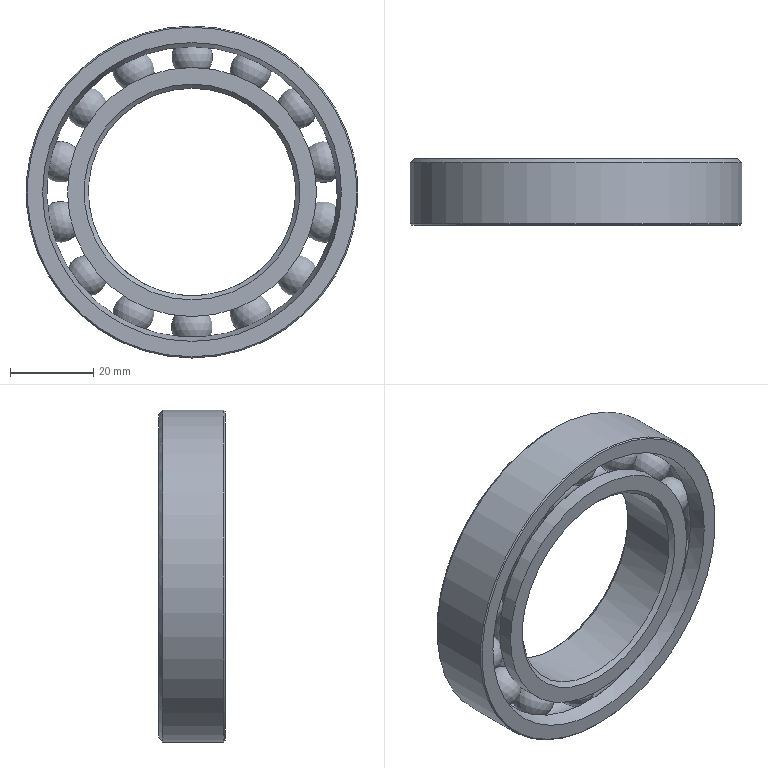Component | NX | BEARING | 16 solids | 30 faces | volume 33031 mm3 | sphere 14 | cylinder 5 | cone 5 | plane 4 | torus 2 | commonest cylinder face diameters 60.001 x2 80 x1 69.999 x1 50 x1